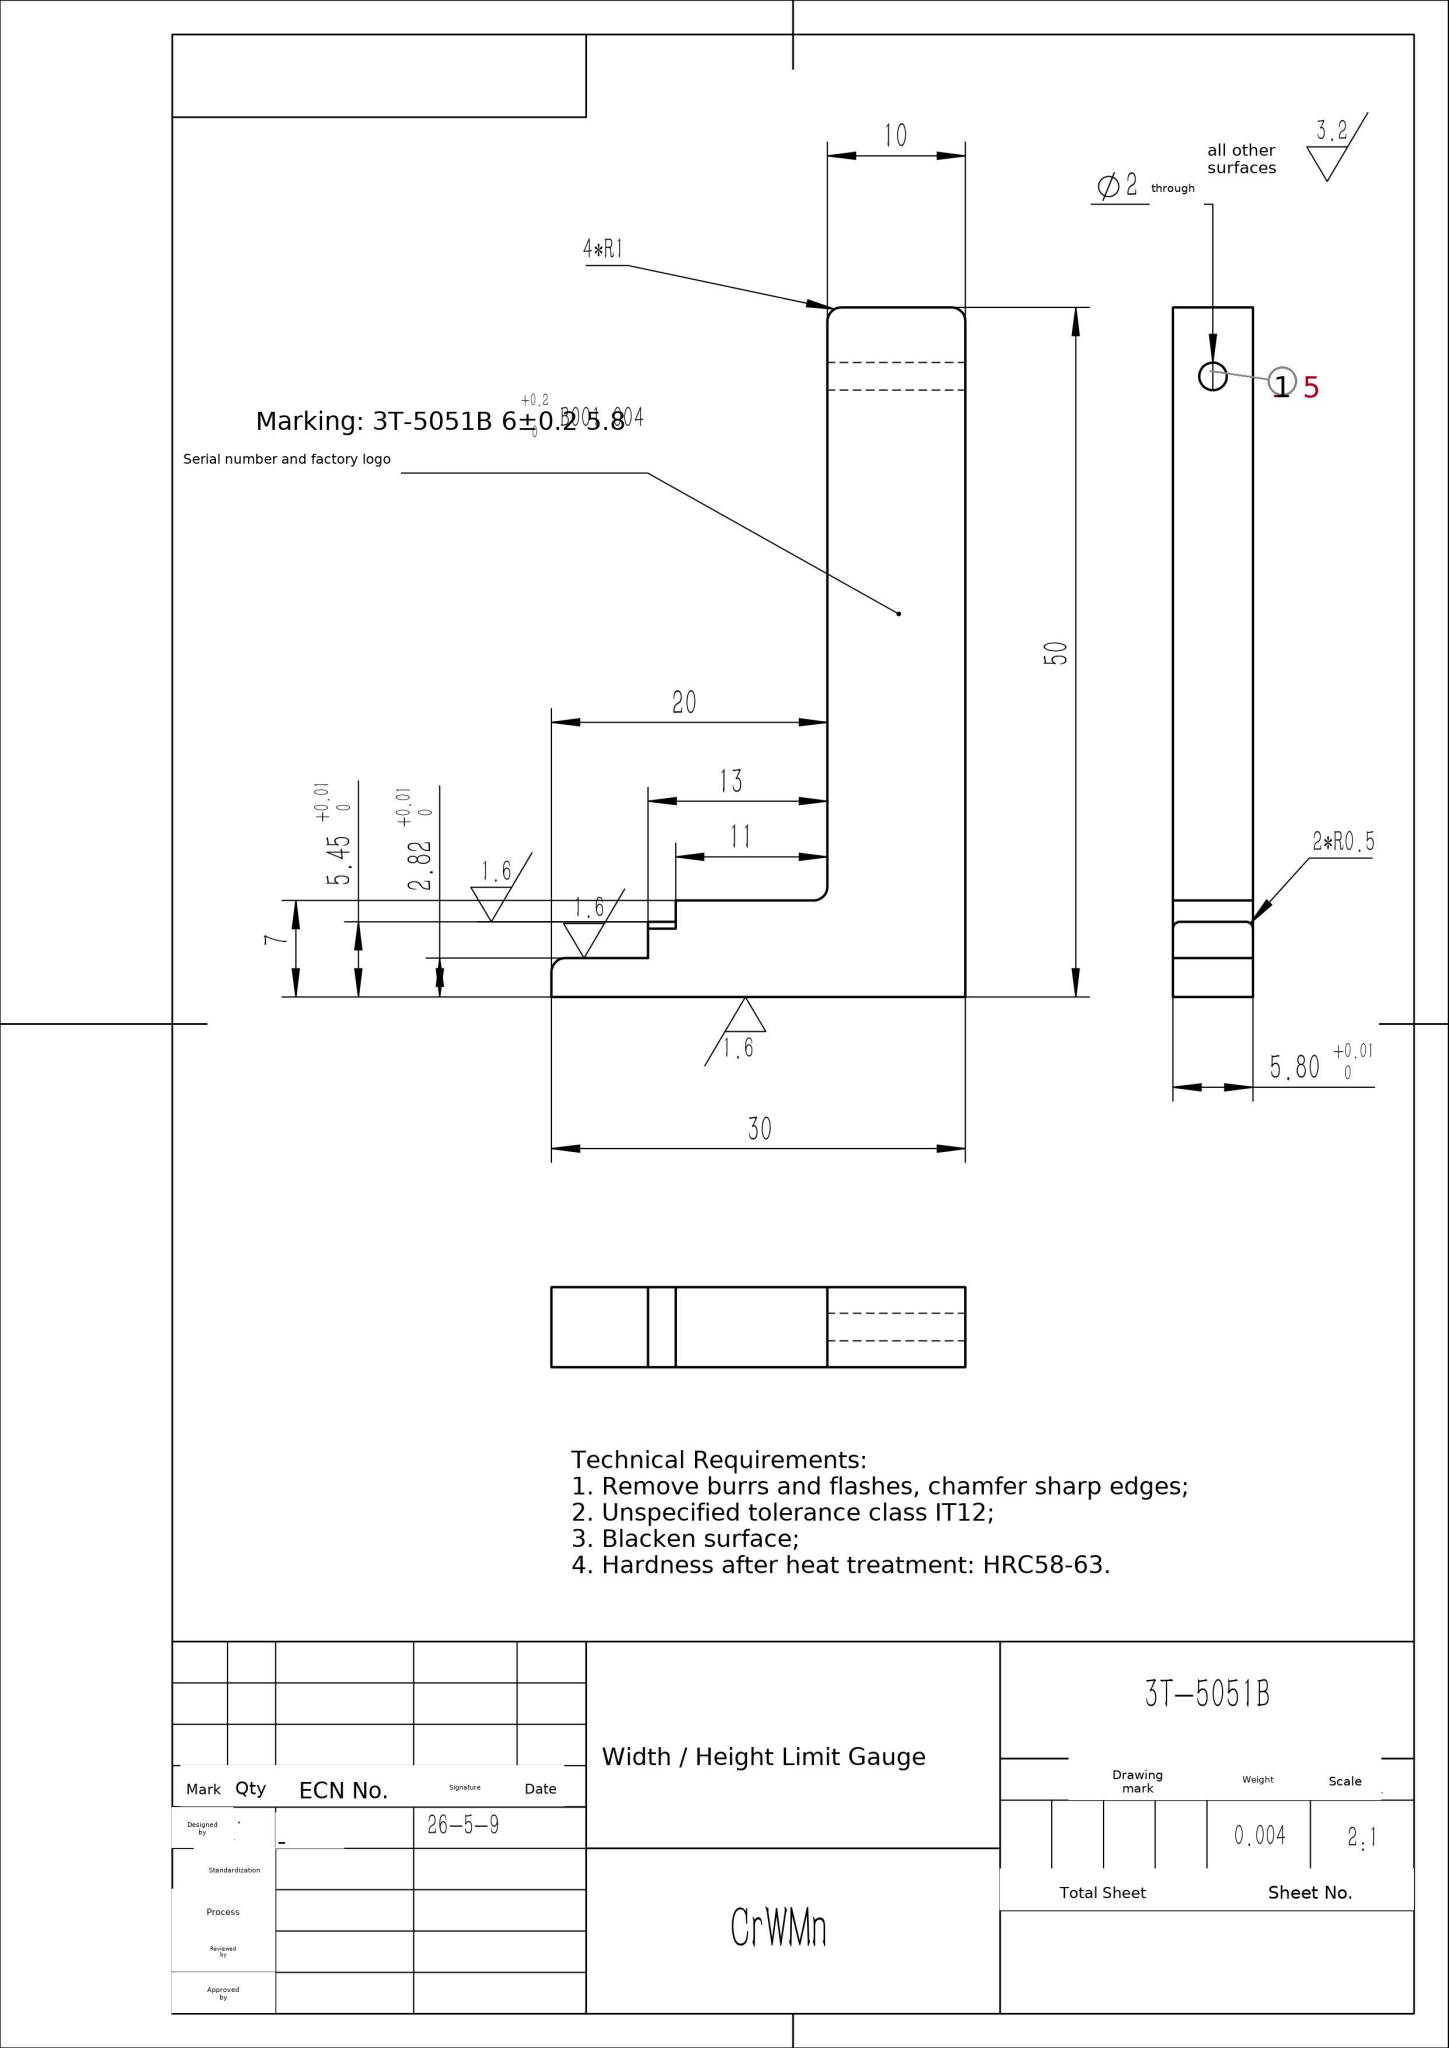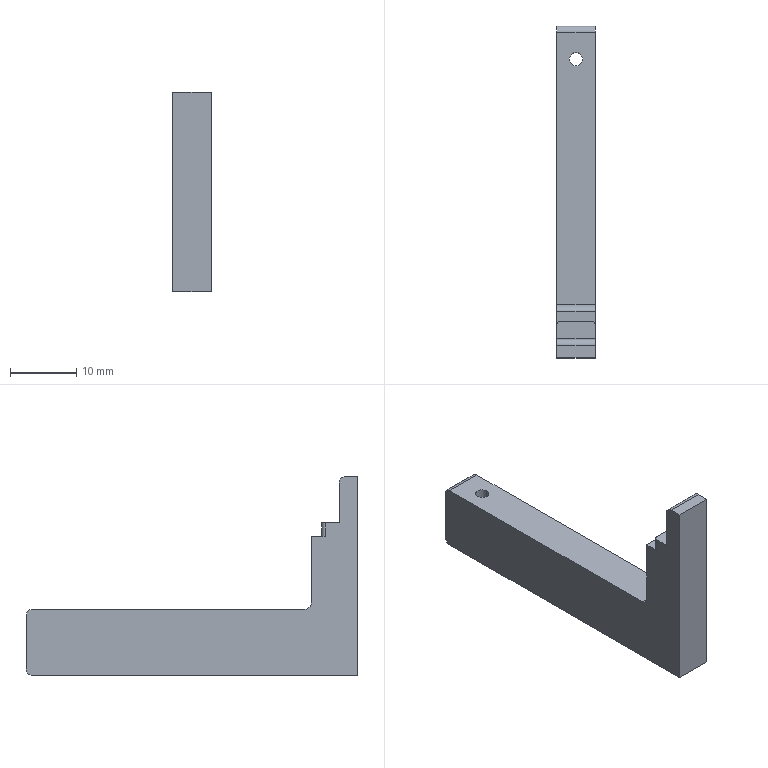Part | SolidWorks | mm | material CrWMn | 1 solid | 20 faces | box 5.8 x 50 x 30 mm | volume 3490 mm3 | plane 12 | cylinder 8 | commonest cylinder face diameters 2 x6 1 x2
STEP:
#1=CARTESIAN_POINT('',(1.,41.5,0.));
#2=VERTEX_POINT('',#1);
#3=CARTESIAN_POINT('',(-1.,41.5,0.));
#4=VERTEX_POINT('',#3);
#5=CARTESIAN_POINT('',(0.,41.5,0.));
#6=DIRECTION('',(0.,0.,-1.));
#7=DIRECTION('',(-1.,0.,0.));
#8=AXIS2_PLACEMENT_3D('',#5,#6,#7);
#9=CIRCLE('',#8,1.);
#10=EDGE_CURVE('',#2,#4,#9,.T.);
#11=ORIENTED_EDGE('',*,*,#10,.F.);
#12=CARTESIAN_POINT('',(1.,41.5,-10.));
#13=VERTEX_POINT('',#12);
#14=CARTESIAN_POINT('',(1.,41.5,20.));
#15=DIRECTION('',(0.,0.,-1.));
#16=VECTOR('',#15,1000.);
#17=LINE('',#14,#16);
#18=EDGE_CURVE('',#2,#13,#17,.T.);
#19=ORIENTED_EDGE('',*,*,#18,.T.);
#20=CARTESIAN_POINT('',(-1.,41.5,-10.));
#21=VERTEX_POINT('',#20);
#22=CARTESIAN_POINT('',(0.,41.5,-10.));
#23=DIRECTION('',(0.,0.,-1.));
#24=DIRECTION('',(-1.,0.,0.));
#25=AXIS2_PLACEMENT_3D('',#22,#23,#24);
#26=CIRCLE('',#25,1.);
#27=EDGE_CURVE('',#13,#21,#26,.T.);
#28=ORIENTED_EDGE('',*,*,#27,.T.);
#29=CARTESIAN_POINT('',(-1.,41.5,20.));
#30=DIRECTION('',(0.,0.,-1.));
#31=VECTOR('',#30,1000.);
#32=LINE('',#29,#31);
#33=EDGE_CURVE('',#4,#21,#32,.T.);
#34=ORIENTED_EDGE('',*,*,#33,.F.);
#35=EDGE_LOOP('',(#11,#19,#28,#34));
#36=FACE_OUTER_BOUND('',#35,.T.);
#37=CARTESIAN_POINT('',(0.,41.5,20.));
#38=DIRECTION('',(0.,0.,-1.));
#39=DIRECTION('',(-1.,0.,0.));
#40=AXIS2_PLACEMENT_3D('',#37,#38,#39);
#41=CYLINDRICAL_SURFACE('',#40,1.);
#42=ADVANCED_FACE('',(#36),#41,.F.);
#43=CARTESIAN_POINT('',(2.9,3.5,11.));
#44=VERTEX_POINT('',#43);
#45=CARTESIAN_POINT('',(2.9,3.5,1.));
#46=VERTEX_POINT('',#45);
#47=CARTESIAN_POINT('',(2.9,3.5,20.));
#48=DIRECTION('',(0.,0.,-1.));
#49=VECTOR('',#48,1000.);
#50=LINE('',#47,#49);
#51=EDGE_CURVE('',#44,#46,#50,.T.);
#52=ORIENTED_EDGE('',*,*,#51,.T.);
#53=CARTESIAN_POINT('',(-2.9,3.5,1.));
#54=VERTEX_POINT('',#53);
#55=CARTESIAN_POINT('',(-2.9,3.5,1.));
#56=DIRECTION('',(-1.,-0.,0.));
#57=VECTOR('',#56,1000.);
#58=LINE('',#55,#57);
#59=EDGE_CURVE('',#46,#54,#58,.T.);
#60=ORIENTED_EDGE('',*,*,#59,.T.);
#61=CARTESIAN_POINT('',(-2.9,3.5,11.));
#62=VERTEX_POINT('',#61);
#63=CARTESIAN_POINT('',(-2.9,3.5,20.));
#64=DIRECTION('',(0.,0.,-1.));
#65=VECTOR('',#64,1000.);
#66=LINE('',#63,#65);
#67=EDGE_CURVE('',#62,#54,#66,.T.);
#68=ORIENTED_EDGE('',*,*,#67,.F.);
#69=CARTESIAN_POINT('',(-2.9,3.5,11.));
#70=DIRECTION('',(-1.,0.,0.));
#71=VECTOR('',#70,1000.);
#72=LINE('',#69,#71);
#73=EDGE_CURVE('',#44,#62,#72,.T.);
#74=ORIENTED_EDGE('',*,*,#73,.F.);
#75=EDGE_LOOP('',(#52,#60,#68,#74));
#76=FACE_OUTER_BOUND('',#75,.T.);
#77=CARTESIAN_POINT('',(2.9,3.5,20.));
#78=DIRECTION('',(0.,-1.,0.));
#79=DIRECTION('',(1.,0.,0.));
#80=AXIS2_PLACEMENT_3D('',#77,#78,#79);
#81=PLANE('',#80);
#82=ADVANCED_FACE('',(#76),#81,.F.);
#83=CARTESIAN_POINT('',(-2.9,1.45,13.));
#84=VERTEX_POINT('',#83);
#85=CARTESIAN_POINT('',(-2.9,-0.68,13.));
#86=VERTEX_POINT('',#85);
#87=CARTESIAN_POINT('',(-2.9,1.95,13.));
#88=DIRECTION('',(0.,-1.,0.));
#89=VECTOR('',#88,1000.);
#90=LINE('',#87,#89);
#91=EDGE_CURVE('',#84,#86,#90,.T.);
#92=ORIENTED_EDGE('',*,*,#91,.F.);
#93=CARTESIAN_POINT('',(-2.9,1.45,11.));
#94=VERTEX_POINT('',#93);
#95=CARTESIAN_POINT('',(-2.9,1.45,20.));
#96=DIRECTION('',(0.,0.,-1.));
#97=VECTOR('',#96,1000.);
#98=LINE('',#95,#97);
#99=EDGE_CURVE('',#84,#94,#98,.T.);
#100=ORIENTED_EDGE('',*,*,#99,.T.);
#101=CARTESIAN_POINT('',(-2.9,3.5,11.));
#102=DIRECTION('',(0.,-1.,0.));
#103=VECTOR('',#102,1000.);
#104=LINE('',#101,#103);
#105=EDGE_CURVE('',#62,#94,#104,.T.);
#106=ORIENTED_EDGE('',*,*,#105,.F.);
#107=ORIENTED_EDGE('',*,*,#67,.T.);
#108=CARTESIAN_POINT('',(-2.9,4.5,0.));
#109=VERTEX_POINT('',#108);
#110=CARTESIAN_POINT('',(-2.9,4.5,1.));
#111=DIRECTION('',(1.,0.,0.));
#112=DIRECTION('',(0.,0.,-1.));
#113=AXIS2_PLACEMENT_3D('',#110,#111,#112);
#114=CIRCLE('',#113,1.);
#115=EDGE_CURVE('',#54,#109,#114,.T.);
#116=ORIENTED_EDGE('',*,*,#115,.T.);
#117=CARTESIAN_POINT('',(-2.9,45.5,0.));
#118=VERTEX_POINT('',#117);
#119=CARTESIAN_POINT('',(-2.9,-3.5,0.));
#120=DIRECTION('',(0.,1.,0.));
#121=VECTOR('',#120,1000.);
#122=LINE('',#119,#121);
#123=EDGE_CURVE('',#109,#118,#122,.T.);
#124=ORIENTED_EDGE('',*,*,#123,.T.);
#125=CARTESIAN_POINT('',(-2.9,46.5,-1.));
#126=VERTEX_POINT('',#125);
#127=CARTESIAN_POINT('',(-2.9,45.5,-1.));
#128=DIRECTION('',(-1.,0.,0.));
#129=DIRECTION('',(0.,0.,-1.));
#130=AXIS2_PLACEMENT_3D('',#127,#128,#129);
#131=CIRCLE('',#130,1.);
#132=EDGE_CURVE('',#118,#126,#131,.T.);
#133=ORIENTED_EDGE('',*,*,#132,.T.);
#134=CARTESIAN_POINT('',(-2.9,46.5,-9.));
#135=VERTEX_POINT('',#134);
#136=CARTESIAN_POINT('',(-2.9,46.5,-10.));
#137=DIRECTION('',(0.,0.,1.));
#138=VECTOR('',#137,1000.);
#139=LINE('',#136,#138);
#140=EDGE_CURVE('',#135,#126,#139,.T.);
#141=ORIENTED_EDGE('',*,*,#140,.F.);
#142=CARTESIAN_POINT('',(-2.9,45.5,-10.));
#143=VERTEX_POINT('',#142);
#144=CARTESIAN_POINT('',(-2.9,45.5,-9.));
#145=DIRECTION('',(-1.,0.,0.));
#146=DIRECTION('',(0.,0.,-1.));
#147=AXIS2_PLACEMENT_3D('',#144,#145,#146);
#148=CIRCLE('',#147,1.);
#149=EDGE_CURVE('',#135,#143,#148,.T.);
#150=ORIENTED_EDGE('',*,*,#149,.T.);
#151=CARTESIAN_POINT('',(-2.9,-3.5,-10.));
#152=VERTEX_POINT('',#151);
#153=CARTESIAN_POINT('',(-2.9,-3.5,-10.));
#154=DIRECTION('',(0.,1.,0.));
#155=VECTOR('',#154,1000.);
#156=LINE('',#153,#155);
#157=EDGE_CURVE('',#152,#143,#156,.T.);
#158=ORIENTED_EDGE('',*,*,#157,.F.);
#159=CARTESIAN_POINT('',(-2.9,-3.5,20.));
#160=VERTEX_POINT('',#159);
#161=CARTESIAN_POINT('',(-2.9,-3.5,20.));
#162=DIRECTION('',(0.,0.,-1.));
#163=VECTOR('',#162,1000.);
#164=LINE('',#161,#163);
#165=EDGE_CURVE('',#160,#152,#164,.T.);
#166=ORIENTED_EDGE('',*,*,#165,.F.);
#167=CARTESIAN_POINT('',(-2.9,-1.68,20.));
#168=VERTEX_POINT('',#167);
#169=CARTESIAN_POINT('',(-2.9,-3.5,20.));
#170=DIRECTION('',(0.,-1.,0.));
#171=VECTOR('',#170,1000.);
#172=LINE('',#169,#171);
#173=EDGE_CURVE('',#168,#160,#172,.T.);
#174=ORIENTED_EDGE('',*,*,#173,.F.);
#175=CARTESIAN_POINT('',(-2.9,-0.68,19.));
#176=VERTEX_POINT('',#175);
#177=CARTESIAN_POINT('',(-2.9,-1.68,19.));
#178=DIRECTION('',(-1.,0.,0.));
#179=DIRECTION('',(0.,0.,-1.));
#180=AXIS2_PLACEMENT_3D('',#177,#178,#179);
#181=CIRCLE('',#180,1.);
#182=EDGE_CURVE('',#168,#176,#181,.T.);
#183=ORIENTED_EDGE('',*,*,#182,.T.);
#184=CARTESIAN_POINT('',(-2.9,-0.68,13.));
#185=DIRECTION('',(0.,0.,1.));
#186=VECTOR('',#185,1000.);
#187=LINE('',#184,#186);
#188=EDGE_CURVE('',#86,#176,#187,.T.);
#189=ORIENTED_EDGE('',*,*,#188,.F.);
#190=EDGE_LOOP('',(#92,#100,#106,#107,#116,#124,#133,#141,#150,#158,#166,#174,#183,#189));
#191=FACE_OUTER_BOUND('',#190,.T.);
#192=CARTESIAN_POINT('',(-2.9,-3.5,20.));
#193=DIRECTION('',(1.,0.,0.));
#194=DIRECTION('',(0.,0.,-1.));
#195=AXIS2_PLACEMENT_3D('',#192,#193,#194);
#196=PLANE('',#195);
#197=ADVANCED_FACE('',(#191),#196,.F.);
#198=ORIENTED_EDGE('',*,*,#165,.T.);
#199=CARTESIAN_POINT('',(2.9,-3.5,-10.));
#200=VERTEX_POINT('',#199);
#201=CARTESIAN_POINT('',(-2.9,-3.5,-10.));
#202=DIRECTION('',(-1.,0.,0.));
#203=VECTOR('',#202,1000.);
#204=LINE('',#201,#203);
#205=EDGE_CURVE('',#200,#152,#204,.T.);
#206=ORIENTED_EDGE('',*,*,#205,.F.);
#207=CARTESIAN_POINT('',(2.9,-3.5,20.));
#208=VERTEX_POINT('',#207);
#209=CARTESIAN_POINT('',(2.9,-3.5,20.));
#210=DIRECTION('',(0.,0.,-1.));
#211=VECTOR('',#210,1000.);
#212=LINE('',#209,#211);
#213=EDGE_CURVE('',#208,#200,#212,.T.);
#214=ORIENTED_EDGE('',*,*,#213,.F.);
#215=CARTESIAN_POINT('',(2.9,-3.5,20.));
#216=DIRECTION('',(1.,0.,0.));
#217=VECTOR('',#216,1000.);
#218=LINE('',#215,#217);
#219=EDGE_CURVE('',#160,#208,#218,.T.);
#220=ORIENTED_EDGE('',*,*,#219,.F.);
#221=EDGE_LOOP('',(#198,#206,#214,#220));
#222=FACE_OUTER_BOUND('',#221,.T.);
#223=CARTESIAN_POINT('',(2.9,-3.5,20.));
#224=DIRECTION('',(-0.,1.,0.));
#225=DIRECTION('',(-1.,-0.,0.));
#226=AXIS2_PLACEMENT_3D('',#223,#224,#225);
#227=PLANE('',#226);
#228=ADVANCED_FACE('',(#222),#227,.F.);
#229=CARTESIAN_POINT('',(2.9,1.45,11.));
#230=VERTEX_POINT('',#229);
#231=CARTESIAN_POINT('',(2.9,3.5,11.));
#232=DIRECTION('',(0.,1.,0.));
#233=VECTOR('',#232,1000.);
#234=LINE('',#231,#233);
#235=EDGE_CURVE('',#230,#44,#234,.T.);
#236=ORIENTED_EDGE('',*,*,#235,.F.);
#237=CARTESIAN_POINT('',(2.9,1.45,13.));
#238=VERTEX_POINT('',#237);
#239=CARTESIAN_POINT('',(2.9,1.45,20.));
#240=DIRECTION('',(0.,0.,1.));
#241=VECTOR('',#240,1000.);
#242=LINE('',#239,#241);
#243=EDGE_CURVE('',#230,#238,#242,.T.);
#244=ORIENTED_EDGE('',*,*,#243,.T.);
#245=CARTESIAN_POINT('',(2.9,-0.68,13.));
#246=VERTEX_POINT('',#245);
#247=CARTESIAN_POINT('',(2.9,-3.5,13.));
#248=DIRECTION('',(0.,1.,0.));
#249=VECTOR('',#248,1000.);
#250=LINE('',#247,#249);
#251=EDGE_CURVE('',#246,#238,#250,.T.);
#252=ORIENTED_EDGE('',*,*,#251,.F.);
#253=CARTESIAN_POINT('',(2.9,-0.68,19.));
#254=VERTEX_POINT('',#253);
#255=CARTESIAN_POINT('',(2.9,-0.68,20.));
#256=DIRECTION('',(0.,0.,1.));
#257=VECTOR('',#256,1000.);
#258=LINE('',#255,#257);
#259=EDGE_CURVE('',#246,#254,#258,.T.);
#260=ORIENTED_EDGE('',*,*,#259,.T.);
#261=CARTESIAN_POINT('',(2.9,-1.68,20.));
#262=VERTEX_POINT('',#261);
#263=CARTESIAN_POINT('',(2.9,-1.68,19.));
#264=DIRECTION('',(1.,0.,0.));
#265=DIRECTION('',(0.,0.,1.));
#266=AXIS2_PLACEMENT_3D('',#263,#264,#265);
#267=CIRCLE('',#266,1.);
#268=EDGE_CURVE('',#254,#262,#267,.T.);
#269=ORIENTED_EDGE('',*,*,#268,.T.);
#270=CARTESIAN_POINT('',(2.9,-3.5,20.));
#271=DIRECTION('',(0.,1.,0.));
#272=VECTOR('',#271,1000.);
#273=LINE('',#270,#272);
#274=EDGE_CURVE('',#208,#262,#273,.T.);
#275=ORIENTED_EDGE('',*,*,#274,.F.);
#276=ORIENTED_EDGE('',*,*,#213,.T.);
#277=CARTESIAN_POINT('',(2.9,45.5,-10.));
#278=VERTEX_POINT('',#277);
#279=CARTESIAN_POINT('',(2.9,-3.5,-10.));
#280=DIRECTION('',(0.,-1.,0.));
#281=VECTOR('',#280,1000.);
#282=LINE('',#279,#281);
#283=EDGE_CURVE('',#278,#200,#282,.T.);
#284=ORIENTED_EDGE('',*,*,#283,.F.);
#285=CARTESIAN_POINT('',(2.9,46.5,-9.));
#286=VERTEX_POINT('',#285);
#287=CARTESIAN_POINT('',(2.9,45.5,-9.));
#288=DIRECTION('',(1.,0.,0.));
#289=DIRECTION('',(0.,0.,1.));
#290=AXIS2_PLACEMENT_3D('',#287,#288,#289);
#291=CIRCLE('',#290,1.);
#292=EDGE_CURVE('',#278,#286,#291,.T.);
#293=ORIENTED_EDGE('',*,*,#292,.T.);
#294=CARTESIAN_POINT('',(2.9,46.5,-1.));
#295=VERTEX_POINT('',#294);
#296=CARTESIAN_POINT('',(2.9,46.5,-10.));
#297=DIRECTION('',(0.,0.,1.));
#298=VECTOR('',#297,1000.);
#299=LINE('',#296,#298);
#300=EDGE_CURVE('',#286,#295,#299,.T.);
#301=ORIENTED_EDGE('',*,*,#300,.T.);
#302=CARTESIAN_POINT('',(2.9,45.5,0.));
#303=VERTEX_POINT('',#302);
#304=CARTESIAN_POINT('',(2.9,45.5,-1.));
#305=DIRECTION('',(1.,0.,0.));
#306=DIRECTION('',(0.,0.,1.));
#307=AXIS2_PLACEMENT_3D('',#304,#305,#306);
#308=CIRCLE('',#307,1.);
#309=EDGE_CURVE('',#295,#303,#308,.T.);
#310=ORIENTED_EDGE('',*,*,#309,.T.);
#311=CARTESIAN_POINT('',(2.9,4.5,0.));
#312=VERTEX_POINT('',#311);
#313=CARTESIAN_POINT('',(2.9,-3.5,0.));
#314=DIRECTION('',(0.,-1.,0.));
#315=VECTOR('',#314,1000.);
#316=LINE('',#313,#315);
#317=EDGE_CURVE('',#303,#312,#316,.T.);
#318=ORIENTED_EDGE('',*,*,#317,.T.);
#319=CARTESIAN_POINT('',(2.9,4.5,1.));
#320=DIRECTION('',(-1.,0.,0.));
#321=DIRECTION('',(0.,0.,1.));
#322=AXIS2_PLACEMENT_3D('',#319,#320,#321);
#323=CIRCLE('',#322,1.);
#324=EDGE_CURVE('',#312,#46,#323,.T.);
#325=ORIENTED_EDGE('',*,*,#324,.T.);
#326=ORIENTED_EDGE('',*,*,#51,.F.);
#327=EDGE_LOOP('',(#236,#244,#252,#260,#269,#275,#276,#284,#293,#301,#310,#318,#325,#326));
#328=FACE_OUTER_BOUND('',#327,.T.);
#329=CARTESIAN_POINT('',(2.9,-3.5,20.));
#330=DIRECTION('',(-1.,0.,0.));
#331=DIRECTION('',(0.,0.,1.));
#332=AXIS2_PLACEMENT_3D('',#329,#330,#331);
#333=PLANE('',#332);
#334=ADVANCED_FACE('',(#328),#333,.F.);
#335=ORIENTED_EDGE('',*,*,#274,.T.);
#336=CARTESIAN_POINT('',(-2.9,-1.68,20.));
#337=DIRECTION('',(-1.,0.,0.));
#338=VECTOR('',#337,1000.);
#339=LINE('',#336,#338);
#340=EDGE_CURVE('',#262,#168,#339,.T.);
#341=ORIENTED_EDGE('',*,*,#340,.T.);
#342=ORIENTED_EDGE('',*,*,#173,.T.);
#343=ORIENTED_EDGE('',*,*,#219,.T.);
#344=EDGE_LOOP('',(#335,#341,#342,#343));
#345=FACE_OUTER_BOUND('',#344,.T.);
#346=CARTESIAN_POINT('',(0.,0.,20.));
#347=DIRECTION('',(0.,0.,1.));
#348=DIRECTION('',(1.,0.,0.));
#349=AXIS2_PLACEMENT_3D('',#346,#347,#348);
#350=PLANE('',#349);
#351=ADVANCED_FACE('',(#345),#350,.T.);
#352=CARTESIAN_POINT('',(2.4,1.95,13.));
#353=VERTEX_POINT('',#352);
#354=CARTESIAN_POINT('',(-2.4,1.95,13.));
#355=VERTEX_POINT('',#354);
#356=CARTESIAN_POINT('',(-2.9,1.95,13.));
#357=DIRECTION('',(-1.,0.,0.));
#358=VECTOR('',#357,1000.);
#359=LINE('',#356,#358);
#360=EDGE_CURVE('',#353,#355,#359,.T.);
#361=ORIENTED_EDGE('',*,*,#360,.T.);
#362=CARTESIAN_POINT('',(-2.4,1.45,13.));
#363=DIRECTION('',(0.,0.,1.));
#364=DIRECTION('',(1.,0.,0.));
#365=AXIS2_PLACEMENT_3D('',#362,#363,#364);
#366=CIRCLE('',#365,0.5);
#367=EDGE_CURVE('',#355,#84,#366,.T.);
#368=ORIENTED_EDGE('',*,*,#367,.T.);
#369=ORIENTED_EDGE('',*,*,#91,.T.);
#370=CARTESIAN_POINT('',(-2.9,-0.68,13.));
#371=DIRECTION('',(1.,0.,0.));
#372=VECTOR('',#371,1000.);
#373=LINE('',#370,#372);
#374=EDGE_CURVE('',#86,#246,#373,.T.);
#375=ORIENTED_EDGE('',*,*,#374,.T.);
#376=ORIENTED_EDGE('',*,*,#251,.T.);
#377=CARTESIAN_POINT('',(2.4,1.45,13.));
#378=DIRECTION('',(0.,0.,1.));
#379=DIRECTION('',(1.,0.,0.));
#380=AXIS2_PLACEMENT_3D('',#377,#378,#379);
#381=CIRCLE('',#380,0.5);
#382=EDGE_CURVE('',#238,#353,#381,.T.);
#383=ORIENTED_EDGE('',*,*,#382,.T.);
#384=EDGE_LOOP('',(#361,#368,#369,#375,#376,#383));
#385=FACE_OUTER_BOUND('',#384,.T.);
#386=CARTESIAN_POINT('',(0.,0.,13.));
#387=DIRECTION('',(0.,0.,1.));
#388=DIRECTION('',(1.,0.,0.));
#389=AXIS2_PLACEMENT_3D('',#386,#387,#388);
#390=PLANE('',#389);
#391=ADVANCED_FACE('',(#385),#390,.T.);
#392=ORIENTED_EDGE('',*,*,#188,.T.);
#393=CARTESIAN_POINT('',(2.9,-0.68,19.));
#394=DIRECTION('',(1.,0.,0.));
#395=VECTOR('',#394,1000.);
#396=LINE('',#393,#395);
#397=EDGE_CURVE('',#176,#254,#396,.T.);
#398=ORIENTED_EDGE('',*,*,#397,.T.);
#399=ORIENTED_EDGE('',*,*,#259,.F.);
#400=ORIENTED_EDGE('',*,*,#374,.F.);
#401=EDGE_LOOP('',(#392,#398,#399,#400));
#402=FACE_OUTER_BOUND('',#401,.T.);
#403=CARTESIAN_POINT('',(-2.9,-0.68,13.));
#404=DIRECTION('',(0.,-1.,0.));
#405=DIRECTION('',(0.,0.,-1.));
#406=AXIS2_PLACEMENT_3D('',#403,#404,#405);
#407=PLANE('',#406);
#408=ADVANCED_FACE('',(#402),#407,.F.);
#409=CARTESIAN_POINT('',(-2.4,1.95,11.));
#410=VERTEX_POINT('',#409);
#411=CARTESIAN_POINT('',(2.4,1.95,11.));
#412=VERTEX_POINT('',#411);
#413=CARTESIAN_POINT('',(-2.9,1.95,11.));
#414=DIRECTION('',(1.,0.,0.));
#415=VECTOR('',#414,1000.);
#416=LINE('',#413,#415);
#417=EDGE_CURVE('',#410,#412,#416,.T.);
#418=ORIENTED_EDGE('',*,*,#417,.F.);
#419=CARTESIAN_POINT('',(-2.4,1.95,11.));
#420=DIRECTION('',(0.,0.,1.));
#421=VECTOR('',#420,1000.);
#422=LINE('',#419,#421);
#423=EDGE_CURVE('',#410,#355,#422,.T.);
#424=ORIENTED_EDGE('',*,*,#423,.T.);
#425=ORIENTED_EDGE('',*,*,#360,.F.);
#426=CARTESIAN_POINT('',(2.4,1.95,11.));
#427=DIRECTION('',(0.,0.,-1.));
#428=VECTOR('',#427,1000.);
#429=LINE('',#426,#428);
#430=EDGE_CURVE('',#353,#412,#429,.T.);
#431=ORIENTED_EDGE('',*,*,#430,.T.);
#432=EDGE_LOOP('',(#418,#424,#425,#431));
#433=FACE_OUTER_BOUND('',#432,.T.);
#434=CARTESIAN_POINT('',(-2.9,1.95,11.));
#435=DIRECTION('',(0.,-1.,0.));
#436=DIRECTION('',(0.,0.,-1.));
#437=AXIS2_PLACEMENT_3D('',#434,#435,#436);
#438=PLANE('',#437);
#439=ADVANCED_FACE('',(#433),#438,.F.);
#440=ORIENTED_EDGE('',*,*,#105,.T.);
#441=CARTESIAN_POINT('',(-2.4,1.45,11.));
#442=DIRECTION('',(0.,0.,-1.));
#443=DIRECTION('',(1.,0.,0.));
#444=AXIS2_PLACEMENT_3D('',#441,#442,#443);
#445=CIRCLE('',#444,0.5);
#446=EDGE_CURVE('',#94,#410,#445,.T.);
#447=ORIENTED_EDGE('',*,*,#446,.T.);
#448=ORIENTED_EDGE('',*,*,#417,.T.);
#449=CARTESIAN_POINT('',(2.4,1.45,11.));
#450=DIRECTION('',(0.,0.,-1.));
#451=DIRECTION('',(1.,0.,0.));
#452=AXIS2_PLACEMENT_3D('',#449,#450,#451);
#453=CIRCLE('',#452,0.5);
#454=EDGE_CURVE('',#412,#230,#453,.T.);
#455=ORIENTED_EDGE('',*,*,#454,.T.);
#456=ORIENTED_EDGE('',*,*,#235,.T.);
#457=ORIENTED_EDGE('',*,*,#73,.T.);
#458=EDGE_LOOP('',(#440,#447,#448,#455,#456,#457));
#459=FACE_OUTER_BOUND('',#458,.T.);
#460=CARTESIAN_POINT('',(0.,0.,11.));
#461=DIRECTION('',(0.,0.,1.));
#462=DIRECTION('',(1.,0.,0.));
#463=AXIS2_PLACEMENT_3D('',#460,#461,#462);
#464=PLANE('',#463);
#465=ADVANCED_FACE('',(#459),#464,.T.);
#466=ORIENTED_EDGE('',*,*,#300,.F.);
#467=CARTESIAN_POINT('',(-2.9,46.5,-9.));
#468=DIRECTION('',(-1.,0.,0.));
#469=VECTOR('',#468,1000.);
#470=LINE('',#467,#469);
#471=EDGE_CURVE('',#286,#135,#470,.T.);
#472=ORIENTED_EDGE('',*,*,#471,.T.);
#473=ORIENTED_EDGE('',*,*,#140,.T.);
#474=CARTESIAN_POINT('',(-2.9,46.5,-1.));
#475=DIRECTION('',(1.,0.,0.));
#476=VECTOR('',#475,1000.);
#477=LINE('',#474,#476);
#478=EDGE_CURVE('',#126,#295,#477,.T.);
#479=ORIENTED_EDGE('',*,*,#478,.T.);
#480=EDGE_LOOP('',(#466,#472,#473,#479));
#481=FACE_OUTER_BOUND('',#480,.T.);
#482=CARTESIAN_POINT('',(-2.9,46.5,-10.));
#483=DIRECTION('',(0.,-1.,0.));
#484=DIRECTION('',(0.,0.,-1.));
#485=AXIS2_PLACEMENT_3D('',#482,#483,#484);
#486=PLANE('',#485);
#487=ADVANCED_FACE('',(#481),#486,.F.);
#488=CARTESIAN_POINT('',(0.,41.5,-10.));
#489=DIRECTION('',(0.,0.,-1.));
#490=DIRECTION('',(-1.,0.,0.));
#491=AXIS2_PLACEMENT_3D('',#488,#489,#490);
#492=CIRCLE('',#491,1.);
#493=EDGE_CURVE('',#21,#13,#492,.T.);
#494=ORIENTED_EDGE('',*,*,#493,.F.);
#495=ORIENTED_EDGE('',*,*,#27,.F.);
#496=EDGE_LOOP('',(#494,#495));
#497=FACE_BOUND('',#496,.T.);
#498=ORIENTED_EDGE('',*,*,#157,.T.);
#499=CARTESIAN_POINT('',(2.9,45.5,-10.));
#500=DIRECTION('',(1.,0.,0.));
#501=VECTOR('',#500,1000.);
#502=LINE('',#499,#501);
#503=EDGE_CURVE('',#143,#278,#502,.T.);
#504=ORIENTED_EDGE('',*,*,#503,.T.);
#505=ORIENTED_EDGE('',*,*,#283,.T.);
#506=ORIENTED_EDGE('',*,*,#205,.T.);
#507=EDGE_LOOP('',(#498,#504,#505,#506));
#508=FACE_OUTER_BOUND('',#507,.T.);
#509=CARTESIAN_POINT('',(0.,0.,-10.));
#510=DIRECTION('',(0.,0.,-1.));
#511=DIRECTION('',(-1.,0.,0.));
#512=AXIS2_PLACEMENT_3D('',#509,#510,#511);
#513=PLANE('',#512);
#514=ADVANCED_FACE('',(#497,#508),#513,.T.);
#515=CARTESIAN_POINT('',(0.,41.5,0.));
#516=DIRECTION('',(0.,0.,-1.));
#517=DIRECTION('',(-1.,0.,0.));
#518=AXIS2_PLACEMENT_3D('',#515,#516,#517);
#519=CIRCLE('',#518,1.);
#520=EDGE_CURVE('',#4,#2,#519,.T.);
#521=ORIENTED_EDGE('',*,*,#520,.T.);
#522=ORIENTED_EDGE('',*,*,#10,.T.);
#523=EDGE_LOOP('',(#521,#522));
#524=FACE_BOUND('',#523,.T.);
#525=ORIENTED_EDGE('',*,*,#317,.F.);
#526=CARTESIAN_POINT('',(0.,45.5,0.));
#527=DIRECTION('',(-1.,0.,0.));
#528=VECTOR('',#527,1000.);
#529=LINE('',#526,#528);
#530=EDGE_CURVE('',#303,#118,#529,.T.);
#531=ORIENTED_EDGE('',*,*,#530,.T.);
#532=ORIENTED_EDGE('',*,*,#123,.F.);
#533=CARTESIAN_POINT('',(2.9,4.5,0.));
#534=DIRECTION('',(1.,0.,0.));
#535=VECTOR('',#534,1000.);
#536=LINE('',#533,#535);
#537=EDGE_CURVE('',#109,#312,#536,.T.);
#538=ORIENTED_EDGE('',*,*,#537,.T.);
#539=EDGE_LOOP('',(#525,#531,#532,#538));
#540=FACE_OUTER_BOUND('',#539,.T.);
#541=CARTESIAN_POINT('',(0.,0.,0.));
#542=DIRECTION('',(0.,0.,-1.));
#543=DIRECTION('',(-1.,0.,0.));
#544=AXIS2_PLACEMENT_3D('',#541,#542,#543);
#545=PLANE('',#544);
#546=ADVANCED_FACE('',(#524,#540),#545,.F.);
#547=ORIENTED_EDGE('',*,*,#182,.F.);
#548=ORIENTED_EDGE('',*,*,#340,.F.);
#549=ORIENTED_EDGE('',*,*,#268,.F.);
#550=ORIENTED_EDGE('',*,*,#397,.F.);
#551=EDGE_LOOP('',(#547,#548,#549,#550));
#552=FACE_OUTER_BOUND('',#551,.T.);
#553=CARTESIAN_POINT('',(-2.9,-1.68,19.));
#554=DIRECTION('',(-1.,0.,0.));
#555=DIRECTION('',(0.,0.,1.));
#556=AXIS2_PLACEMENT_3D('',#553,#554,#555);
#557=CYLINDRICAL_SURFACE('',#556,1.);
#558=ADVANCED_FACE('',(#552),#557,.T.);
#559=ORIENTED_EDGE('',*,*,#149,.F.);
#560=ORIENTED_EDGE('',*,*,#471,.F.);
#561=ORIENTED_EDGE('',*,*,#292,.F.);
#562=ORIENTED_EDGE('',*,*,#503,.F.);
#563=EDGE_LOOP('',(#559,#560,#561,#562));
#564=FACE_OUTER_BOUND('',#563,.T.);
#565=CARTESIAN_POINT('',(0.,45.5,-9.));
#566=DIRECTION('',(-1.,0.,0.));
#567=DIRECTION('',(0.,0.,1.));
#568=AXIS2_PLACEMENT_3D('',#565,#566,#567);
#569=CYLINDRICAL_SURFACE('',#568,1.);
#570=ADVANCED_FACE('',(#564),#569,.T.);
#571=ORIENTED_EDGE('',*,*,#132,.F.);
#572=ORIENTED_EDGE('',*,*,#530,.F.);
#573=ORIENTED_EDGE('',*,*,#309,.F.);
#574=ORIENTED_EDGE('',*,*,#478,.F.);
#575=EDGE_LOOP('',(#571,#572,#573,#574));
#576=FACE_OUTER_BOUND('',#575,.T.);
#577=CARTESIAN_POINT('',(-2.9,45.5,-1.));
#578=DIRECTION('',(1.,0.,0.));
#579=DIRECTION('',(0.,0.,-1.));
#580=AXIS2_PLACEMENT_3D('',#577,#578,#579);
#581=CYLINDRICAL_SURFACE('',#580,1.);
#582=ADVANCED_FACE('',(#576),#581,.T.);
#583=ORIENTED_EDGE('',*,*,#324,.F.);
#584=ORIENTED_EDGE('',*,*,#537,.F.);
#585=ORIENTED_EDGE('',*,*,#115,.F.);
#586=ORIENTED_EDGE('',*,*,#59,.F.);
#587=EDGE_LOOP('',(#583,#584,#585,#586));
#588=FACE_OUTER_BOUND('',#587,.T.);
#589=CARTESIAN_POINT('',(2.9,4.5,1.));
#590=DIRECTION('',(1.,0.,0.));
#591=DIRECTION('',(0.,1.,0.));
#592=AXIS2_PLACEMENT_3D('',#589,#590,#591);
#593=CYLINDRICAL_SURFACE('',#592,1.);
#594=ADVANCED_FACE('',(#588),#593,.F.);
#595=ORIENTED_EDGE('',*,*,#18,.F.);
#596=ORIENTED_EDGE('',*,*,#520,.F.);
#597=ORIENTED_EDGE('',*,*,#33,.T.);
#598=ORIENTED_EDGE('',*,*,#493,.T.);
#599=EDGE_LOOP('',(#595,#596,#597,#598));
#600=FACE_OUTER_BOUND('',#599,.T.);
#601=CARTESIAN_POINT('',(0.,41.5,20.));
#602=DIRECTION('',(0.,0.,-1.));
#603=DIRECTION('',(-1.,0.,0.));
#604=AXIS2_PLACEMENT_3D('',#601,#602,#603);
#605=CYLINDRICAL_SURFACE('',#604,1.);
#606=ADVANCED_FACE('',(#600),#605,.F.);
#607=ORIENTED_EDGE('',*,*,#446,.F.);
#608=ORIENTED_EDGE('',*,*,#99,.F.);
#609=ORIENTED_EDGE('',*,*,#367,.F.);
#610=ORIENTED_EDGE('',*,*,#423,.F.);
#611=EDGE_LOOP('',(#607,#608,#609,#610));
#612=FACE_OUTER_BOUND('',#611,.T.);
#613=CARTESIAN_POINT('',(-2.4,1.45,11.));
#614=DIRECTION('',(0.,0.,1.));
#615=DIRECTION('',(1.,0.,0.));
#616=AXIS2_PLACEMENT_3D('',#613,#614,#615);
#617=CYLINDRICAL_SURFACE('',#616,0.5);
#618=ADVANCED_FACE('',(#612),#617,.T.);
#619=ORIENTED_EDGE('',*,*,#454,.F.);
#620=ORIENTED_EDGE('',*,*,#430,.F.);
#621=ORIENTED_EDGE('',*,*,#382,.F.);
#622=ORIENTED_EDGE('',*,*,#243,.F.);
#623=EDGE_LOOP('',(#619,#620,#621,#622));
#624=FACE_OUTER_BOUND('',#623,.T.);
#625=CARTESIAN_POINT('',(2.4,1.45,20.));
#626=DIRECTION('',(0.,0.,1.));
#627=DIRECTION('',(1.,0.,0.));
#628=AXIS2_PLACEMENT_3D('',#625,#626,#627);
#629=CYLINDRICAL_SURFACE('',#628,0.5);
#630=ADVANCED_FACE('',(#624),#629,.T.);
#631=CLOSED_SHELL('',(#42,#82,#197,#228,#334,#351,#391,#408,#439,#465,#487,#514,#546,#558,#570,#582,#594,#606,#618,#630));
#632=MANIFOLD_SOLID_BREP('',#631);
#633=CARTESIAN_POINT('',(0.,0.,0.));
#634=DIRECTION('',(0.,0.,1.));
#635=DIRECTION('',(1.,0.,0.));
#636=AXIS2_PLACEMENT_3D('',#633,#634,#635);
#637=(LENGTH_UNIT()NAMED_UNIT(*)SI_UNIT(.MILLI.,.METRE.));
#638=UNCERTAINTY_MEASURE_WITH_UNIT(LENGTH_MEASURE(0.00001),#637,'','');
#639=(NAMED_UNIT(*)PLANE_ANGLE_UNIT()SI_UNIT($,.RADIAN.));
#640=(NAMED_UNIT(*)SI_UNIT($,.STERADIAN.)SOLID_ANGLE_UNIT());
#641=(GEOMETRIC_REPRESENTATION_CONTEXT(3)GLOBAL_UNCERTAINTY_ASSIGNED_CONTEXT((#638))GLOBAL_UNIT_ASSIGNED_CONTEXT((#637,#639,#640))REPRESENTATION_CONTEXT('',''));
#642=ADVANCED_BREP_SHAPE_REPRESENTATION('',(#632,#636),#641);